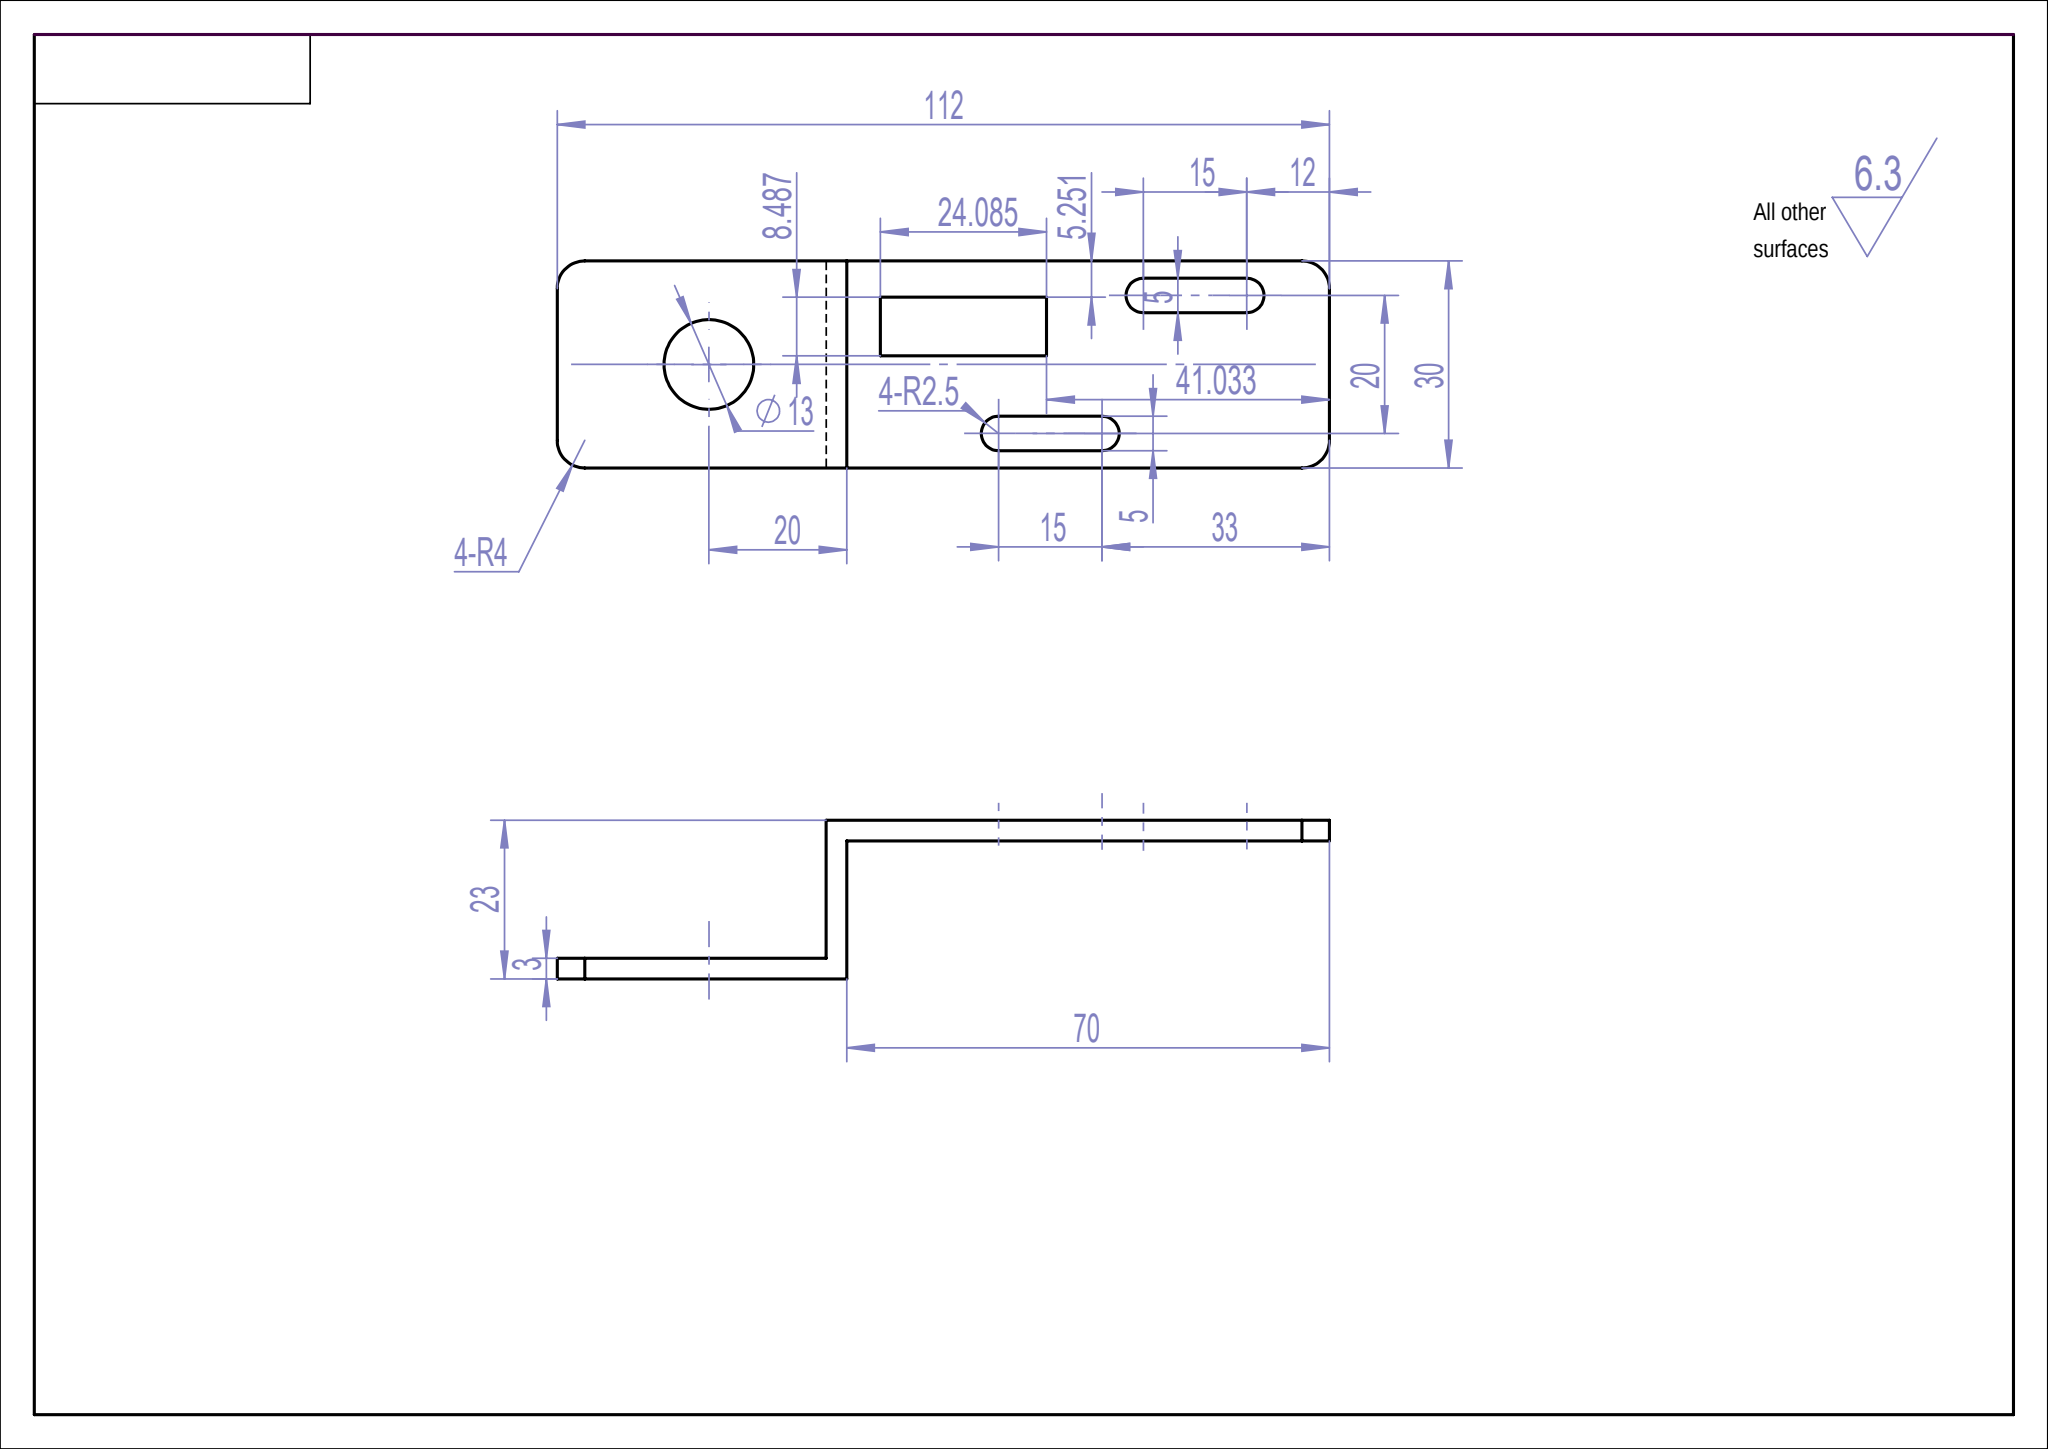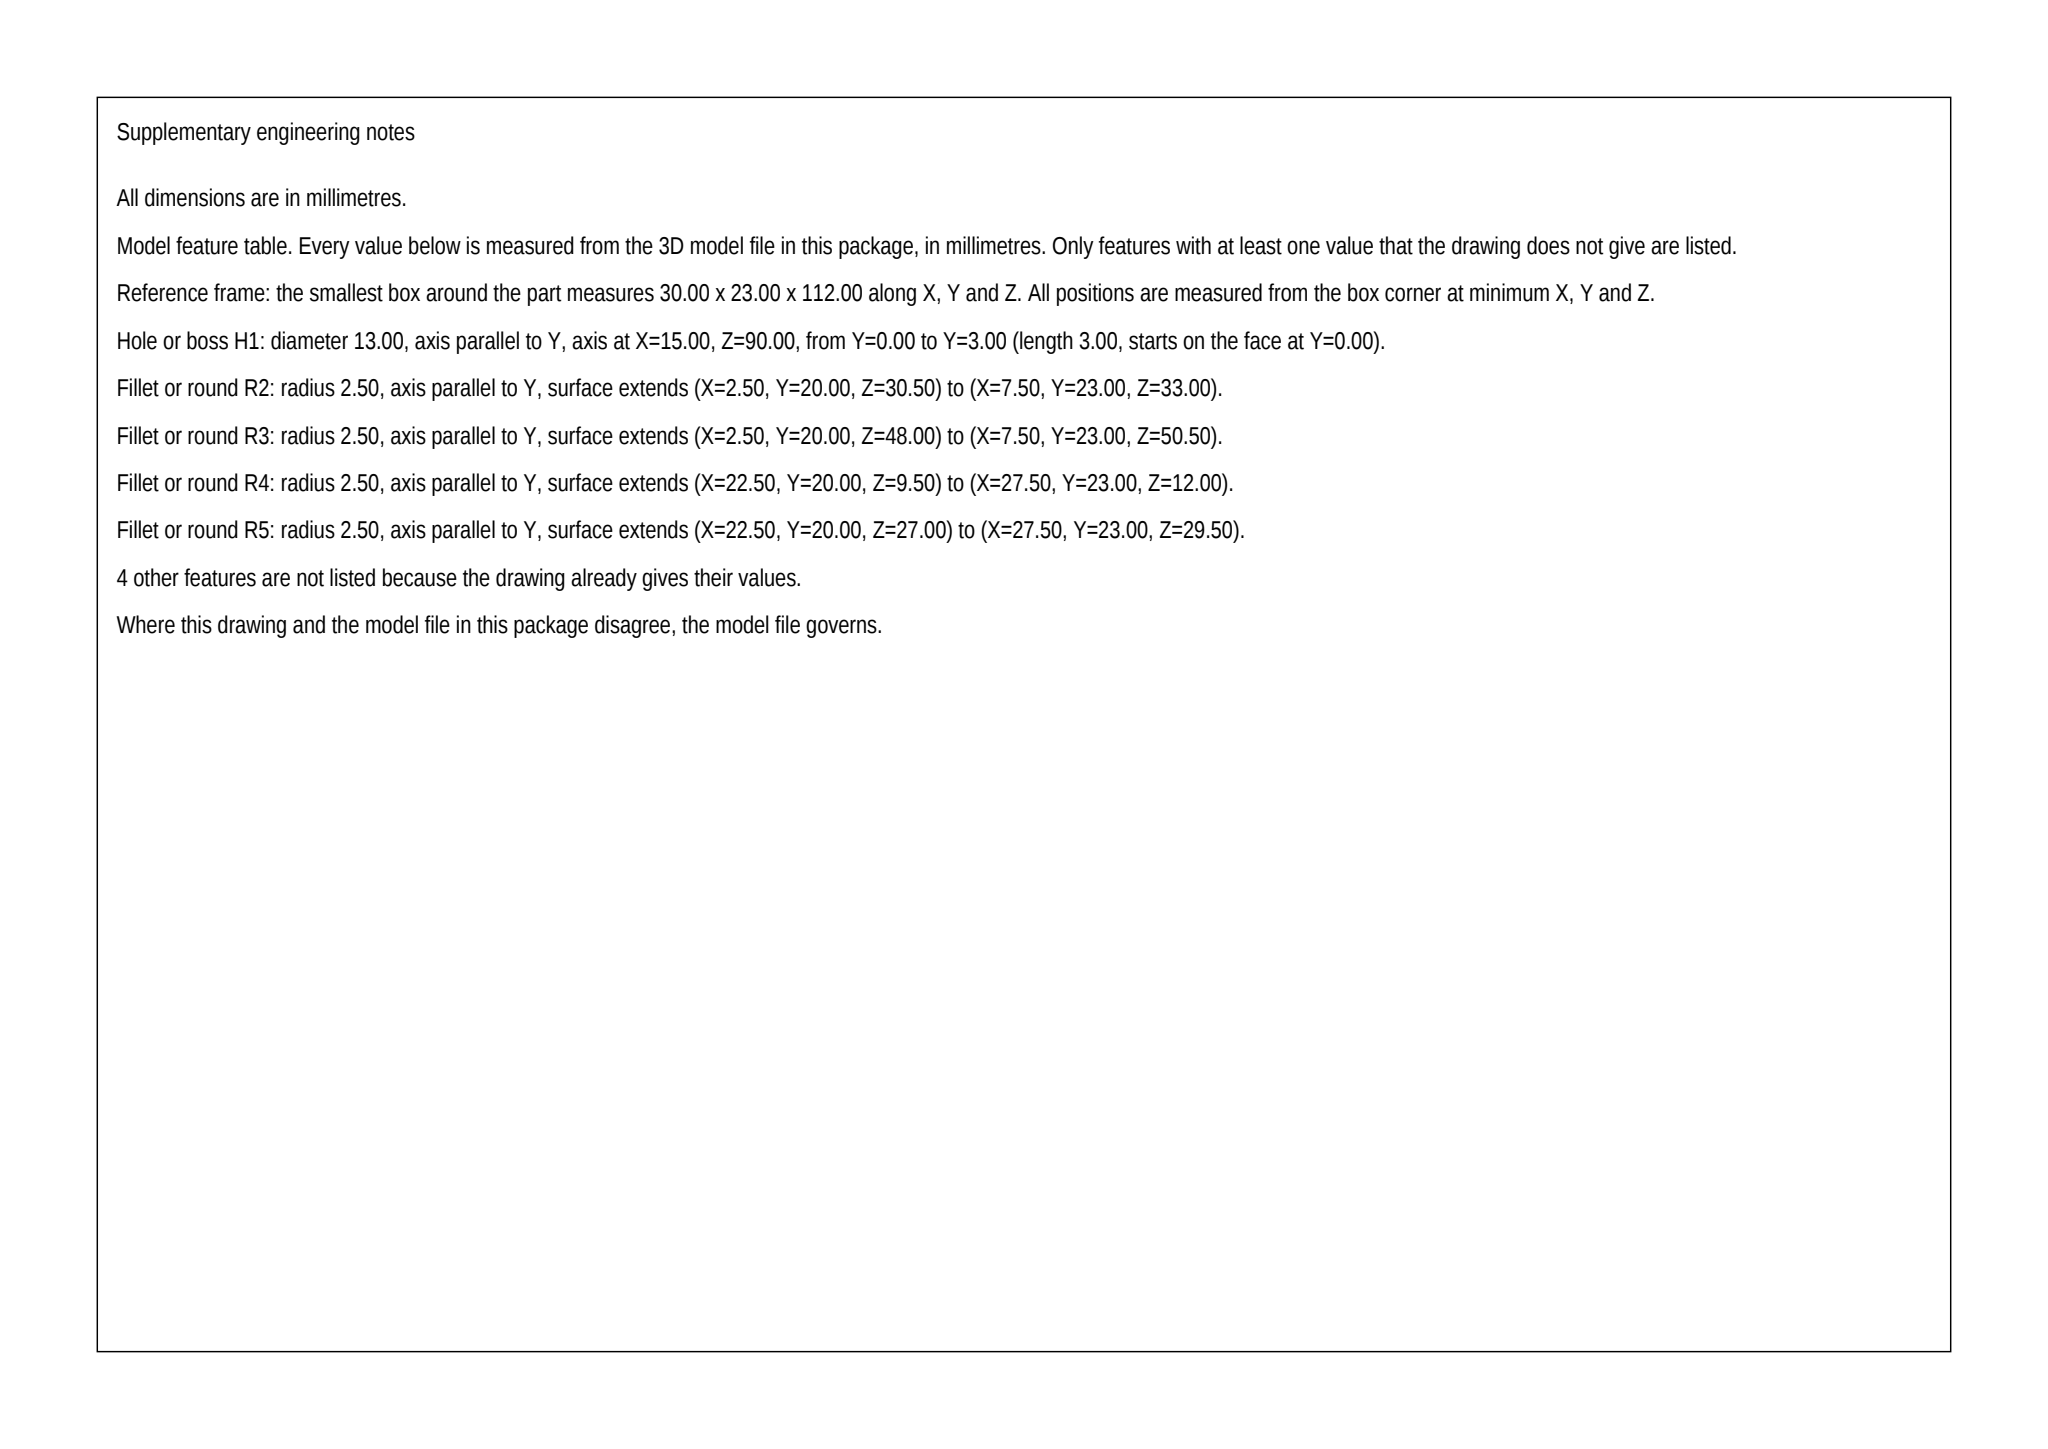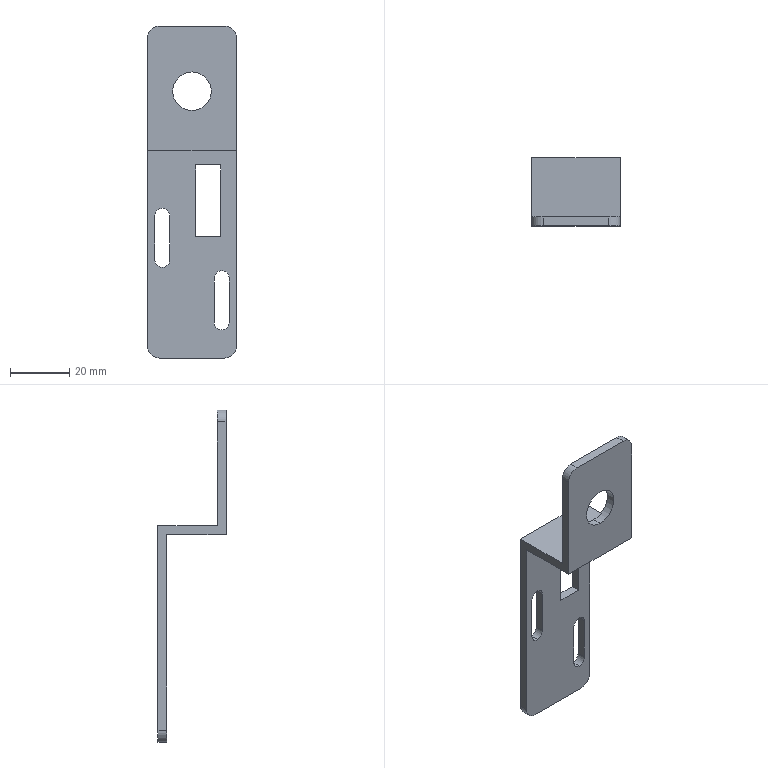Part | SolidWorks | mm | 1 solid | 30 faces | box 30 x 23 x 112 mm | volume 10260 mm3 | plane 18 | cylinder 12 | commonest cylinder face diameters 5 x6 8 x4 13 x2
build123d program:
from build123d import *

# Parameters (mm, degrees)
BOSS_EXTRUDE1_DEPTH = 15
SKETCH2_R           = 6.5
CUT_EXTRUDE1_DEPTH  = 78.994
CUT_EXTRUDE2_REACH  = 79.162
FILLET1_R           = 4
SKETCH4_W           = 8.487
SKETCH4_H           = 24.085
CUT_EXTRUDE3_DEPTH  = 10


with BuildPart() as part:
    # Sketch1 → Boss-Extrude1 (new, symmetric)
    with BuildSketch(Plane(origin=(0, 0, 0), x_dir=(0, 0, -1), z_dir=(1, 0, 0))):
        Polygon((0, 0), (73, 0), (73, -3), (3, -3), (3, -23), (-39, -23), (-39, -20), (0, -20), align=None)
    extrude(amount=BOSS_EXTRUDE1_DEPTH, both=True)

    # Sketch2 → Cut-Extrude1 (cut, through all)
    with BuildSketch(Plane.XZ.offset(23)):
        with Locations(Location((0, 17, 0), (0, 0, 270))):
            Circle(SKETCH2_R)
    extrude(amount=-CUT_EXTRUDE1_DEPTH, mode=Mode.SUBTRACT)

    # Sketch3 → Cut-Extrude2 (cut, up to next)
    with BuildSketch(Plane.XZ.offset(3), mode=Mode.PRIVATE) as cut_extrude2_sk1:
        with BuildLine():
            Line((12.5, -46), (12.5, -61))
            ThreePointArc((12.5, -61), (10, -63.5), (7.5, -61))
            Line((7.5, -61), (7.5, -46))
            ThreePointArc((7.5, -46), (10, -43.5), (12.5, -46))
        make_face()
    cut_extrude2_tool1 = extrude(cut_extrude2_sk1.sketch, amount=-CUT_EXTRUDE2_REACH, mode=Mode.PRIVATE) & part.part
    # Sketch3 → Cut-Extrude2 (cut, up to next)
    with BuildSketch(Plane.XZ.offset(3), mode=Mode.PRIVATE) as cut_extrude2_sk2:
        with BuildLine():
            Line((-7.5, -25), (-7.5, -40))
            ThreePointArc((-7.5, -40), (-10, -42.5), (-12.5, -40))
            Line((-12.5, -40), (-12.5, -25))
            ThreePointArc((-12.5, -25), (-10, -22.5), (-7.5, -25))
        make_face()
    cut_extrude2_tool2 = extrude(cut_extrude2_sk2.sketch, amount=-CUT_EXTRUDE2_REACH, mode=Mode.PRIVATE) & part.part
    add(cut_extrude2_tool1.solids().sort_by_distance((10, -3, -53.5))[0], mode=Mode.SUBTRACT)
    add(cut_extrude2_tool2.solids().sort_by_distance((-10, -3, -32.5))[0], mode=Mode.SUBTRACT)

    # Fillet1
    fillet1_edges = [part.edges().sort_by_distance(p)[0] for p in [
        (15, -21.5, 39),
        (15, -1.5, -73),
        (-15, -1.5, -73),
        (-15, -21.5, 39),
    ]]
    fillet(fillet1_edges, radius=FILLET1_R)

    # Sketch4 → Cut-Extrude3 (cut)
    with BuildSketch(Plane(origin=(0, 0, 0), x_dir=(1, 0, 0), z_dir=(0, 1, 0))):
        with Locations((5.505, 19.925)):
            Rectangle(SKETCH4_W, SKETCH4_H)
    extrude(amount=-CUT_EXTRUDE3_DEPTH, mode=Mode.SUBTRACT)


solid = part.part